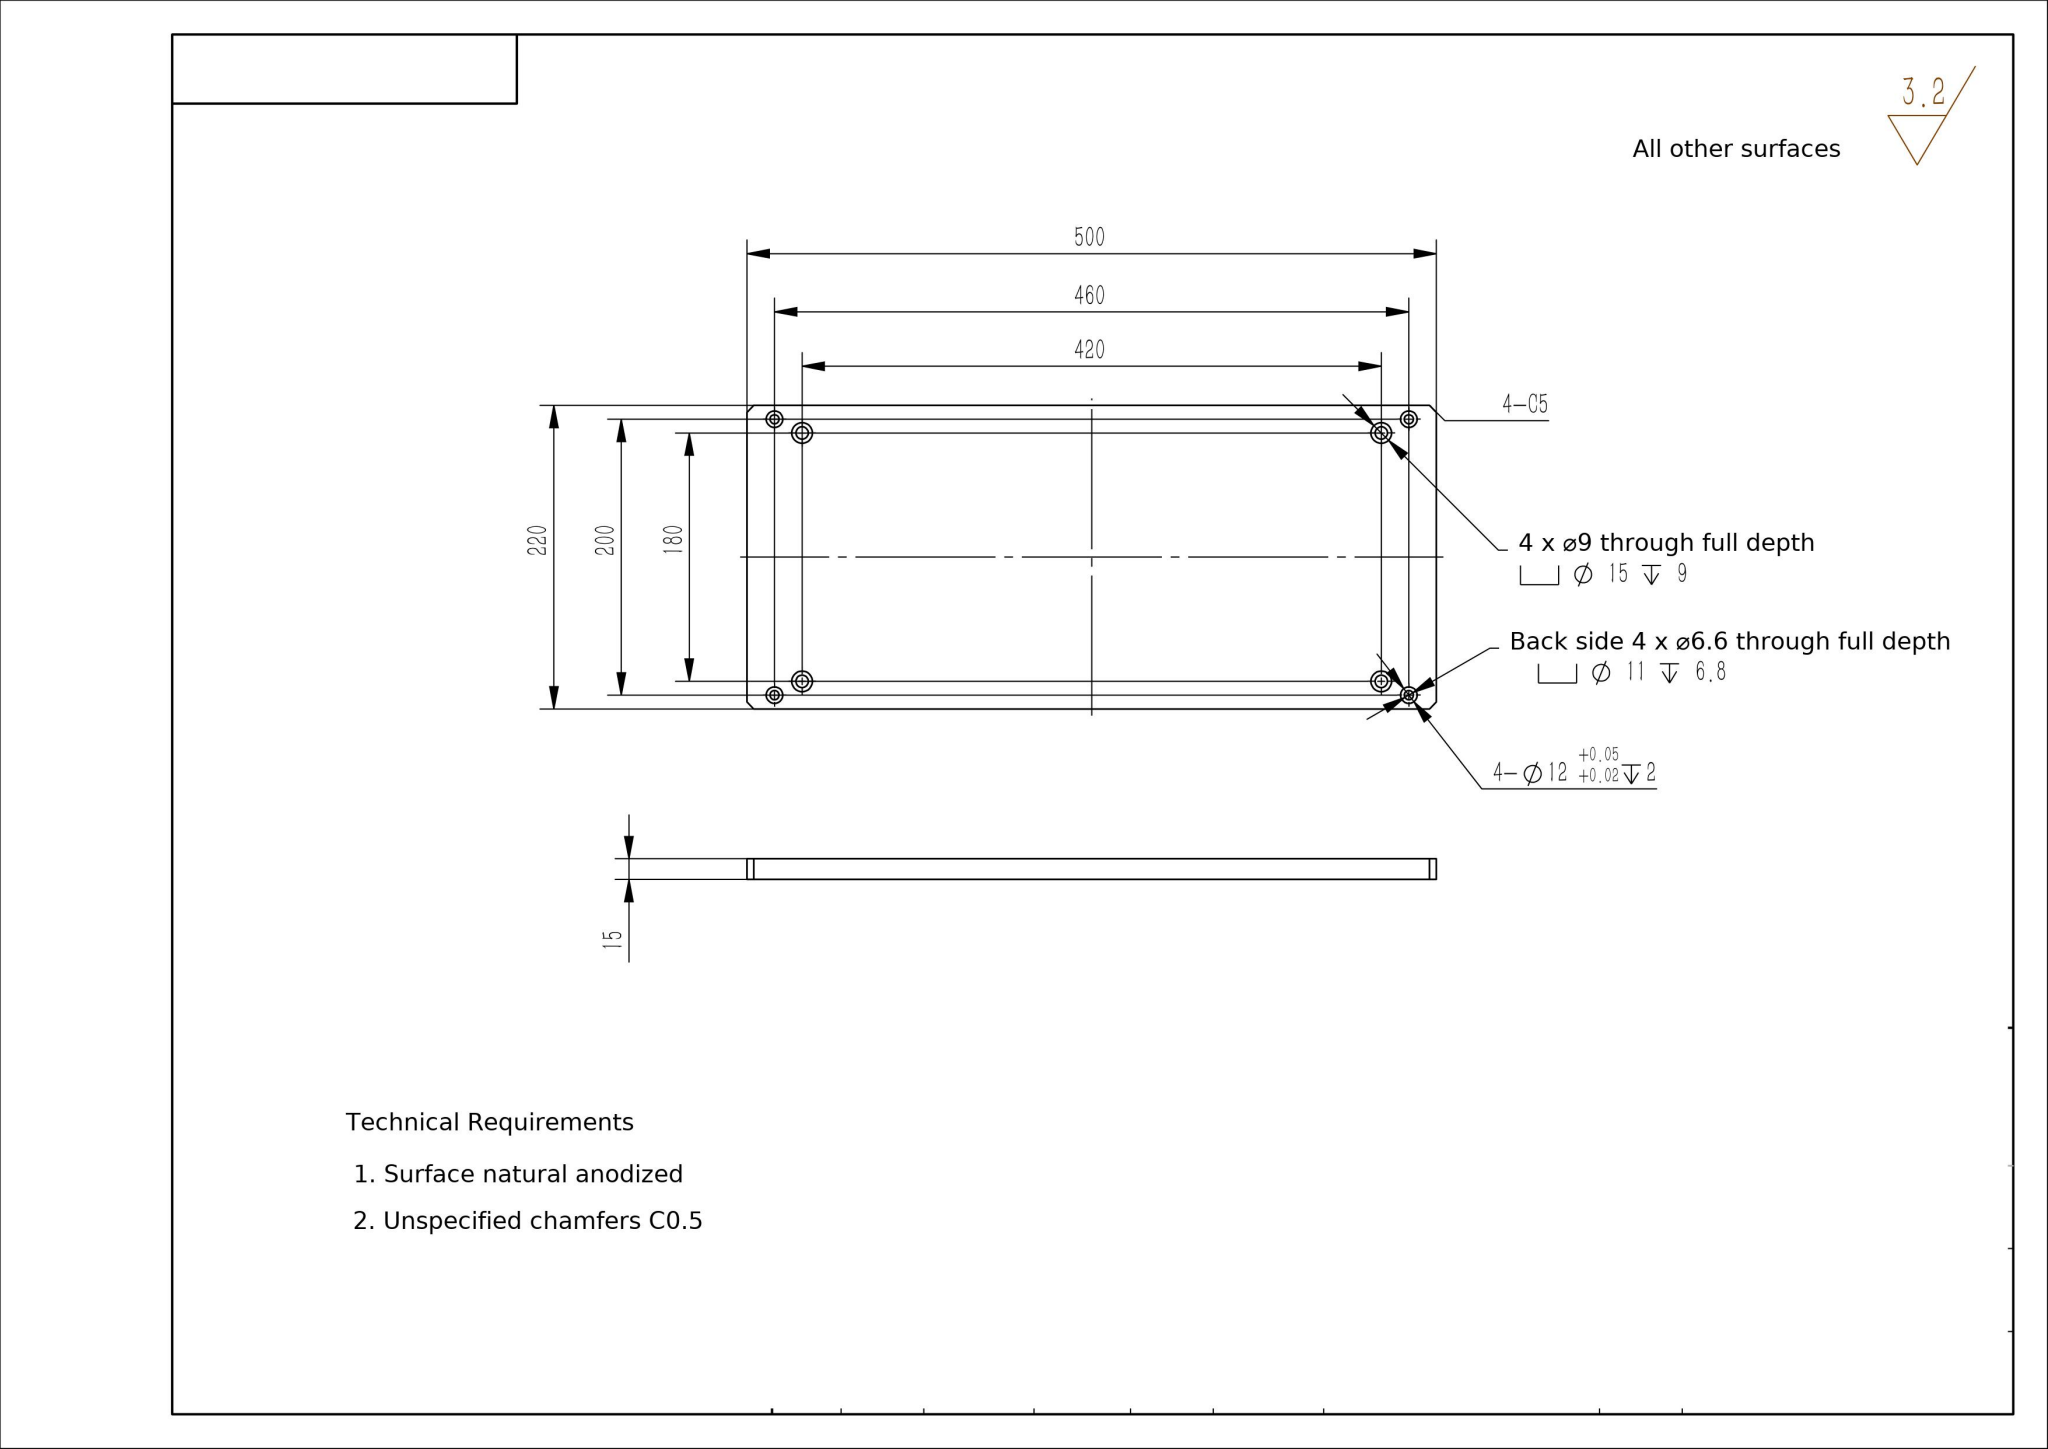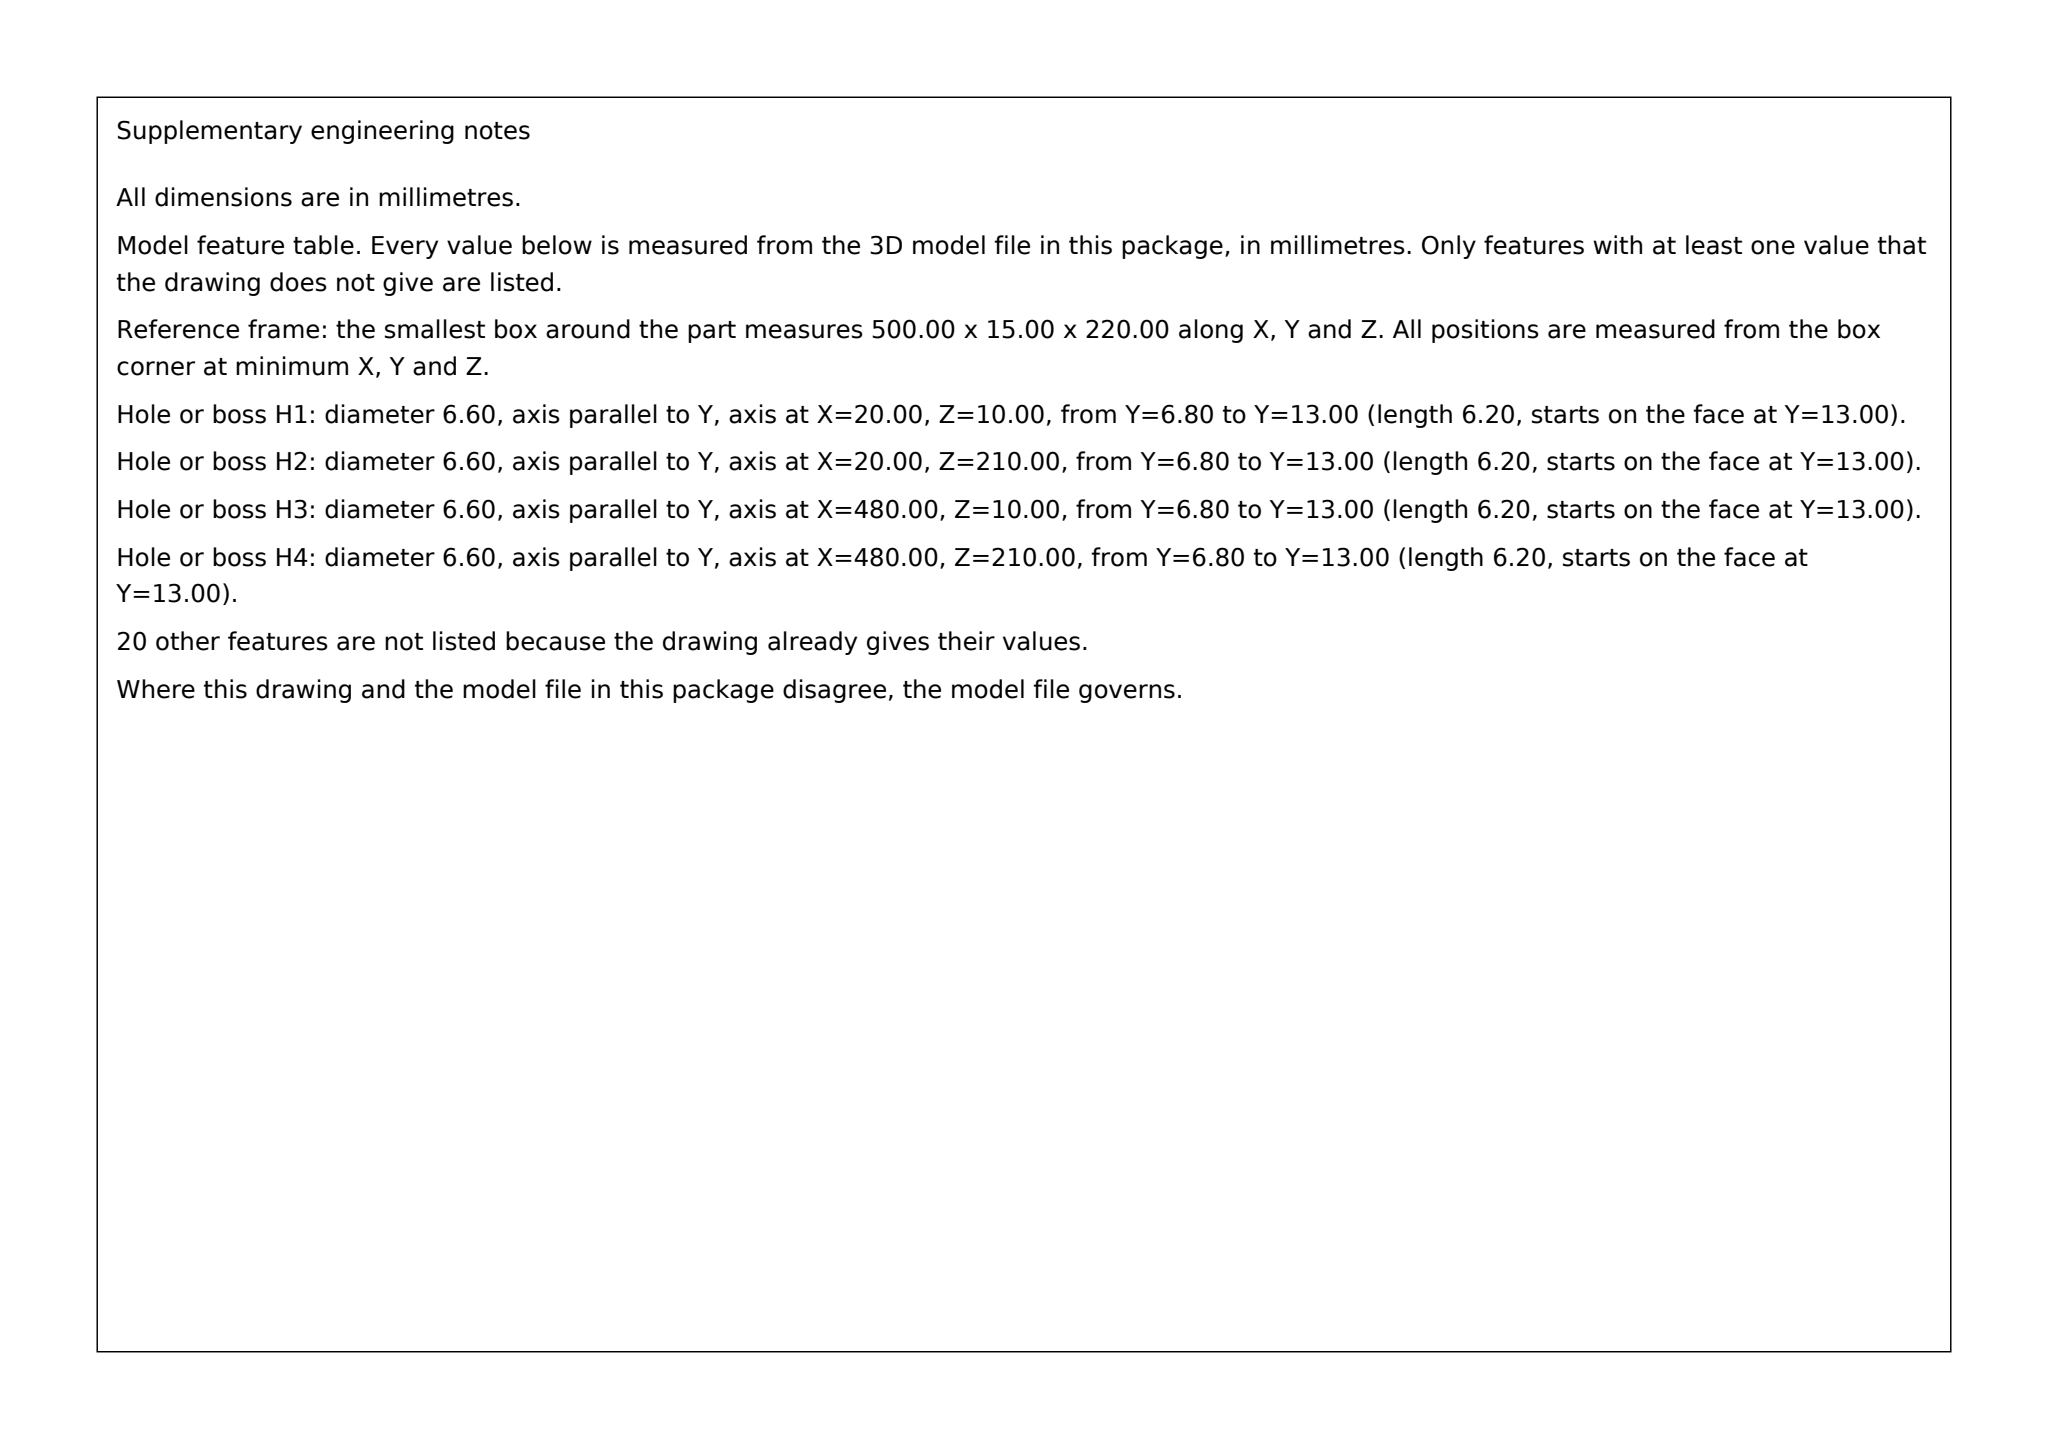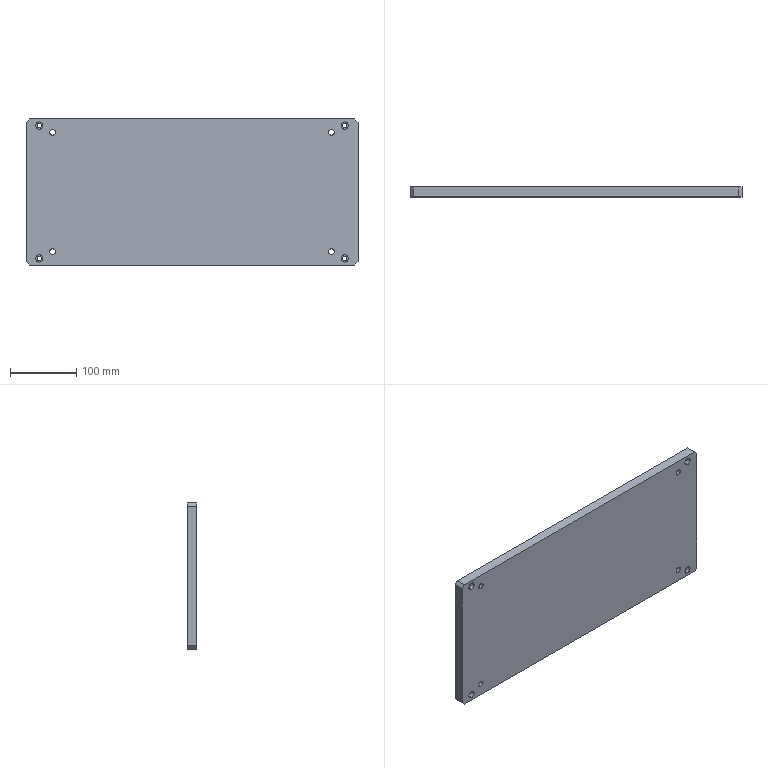Part | SolidWorks | mm | 1 solid | 62 faces | box 500 x 15 x 220 mm | volume 1637023 mm3 | cylinder 40 | plane 22 | commonest cylinder face diameters 15 x8 9 x8 11 x8 6.6 x8 12 x8
build123d program:
from build123d import *

# Parameters (mm, degrees)
SKETCH1_W                                         = 500
SKETCH1_H                                         = 220
BOSS_EXTRUDE1_DEPTH                               = 15
CHAMFER1_SIZE                                     = 5
SKETCH2_R                                         = 6
CUT_EXTRUDE1_DEPTH                                = 2
HOLE_SIZE_ACCORDING_TO_HEXAGON_SOCKET_D           = 6.6
HOLE_SIZE_ACCORDING_TO_HEXAGON_SOCKET_CBORE_D     = 11
HOLE_SIZE_ACCORDING_TO_HEXAGON_SOCKET_CBORE_DEPTH = 6.8
HOLE_SIZE_ACCORDING_TO_HEXAGON_SO_2_D             = 9
HOLE_SIZE_ACCORDING_TO_HEXAGON_SO_2_CBORE_D       = 15
HOLE_SIZE_ACCORDING_TO_HEXAGON_SO_2_CBORE_DEPTH   = 9


with BuildPart() as part:
    # Sketch1 → Boss-Extrude1 (new body)
    with BuildSketch(Plane(origin=(0, 0, 0), x_dir=(1, 0, 0), z_dir=(0, 1, 0))):
        Rectangle(SKETCH1_W, SKETCH1_H)
    extrude(amount=BOSS_EXTRUDE1_DEPTH)

    # Chamfer1
    chamfer1_edges = [part.edges().sort_by_distance(p)[0] for p in [
        (250, 7.5, 110),
        (-250, 7.5, 110),
        (-250, 7.5, -110),
        (250, 7.5, -110),
    ]]
    chamfer(chamfer1_edges, length=CHAMFER1_SIZE)

    # Sketch2 → Cut-Extrude1 (cut)
    with BuildSketch(Plane(origin=(0, 15, 0), x_dir=(1, 0, 0), z_dir=(0, 1, 0))):
        with Locations(Location((-230, 100, 0), (0, 0, 270))):
            Circle(SKETCH2_R)
        with Locations(Location((230, 100, 0), (0, 0, 270))):
            Circle(SKETCH2_R)
        with Locations(Location((-230, -100, 0), (0, 0, 270))):
            Circle(SKETCH2_R)
        with Locations(Location((230, -100, 0), (0, 0, 270))):
            Circle(SKETCH2_R)
    extrude(amount=-CUT_EXTRUDE1_DEPTH, mode=Mode.SUBTRACT)

    # Hole Size _ according to_ Hexagon Socket (through all)
    with Locations(Plane(origin=(0, 0, 0), x_dir=(-1, 0, 0), z_dir=(0, -1, 0))):
        with Locations((-230, 100), (-230, -100), (230, 100), (230, -100)):
            CounterBoreHole(HOLE_SIZE_ACCORDING_TO_HEXAGON_SOCKET_D / 2, HOLE_SIZE_ACCORDING_TO_HEXAGON_SOCKET_CBORE_D / 2, HOLE_SIZE_ACCORDING_TO_HEXAGON_SOCKET_CBORE_DEPTH)

    # Hole Size _ according to_ Hexagon So 2 (through all)
    with Locations(Plane(origin=(0, 15, 0), x_dir=(1, 0, 0), z_dir=(0, 1, 0))):
        with Locations((210, 90), (210, -90), (-210, -90), (-210, 90)):
            CounterBoreHole(HOLE_SIZE_ACCORDING_TO_HEXAGON_SO_2_D / 2, HOLE_SIZE_ACCORDING_TO_HEXAGON_SO_2_CBORE_D / 2, HOLE_SIZE_ACCORDING_TO_HEXAGON_SO_2_CBORE_DEPTH)


solid = part.part